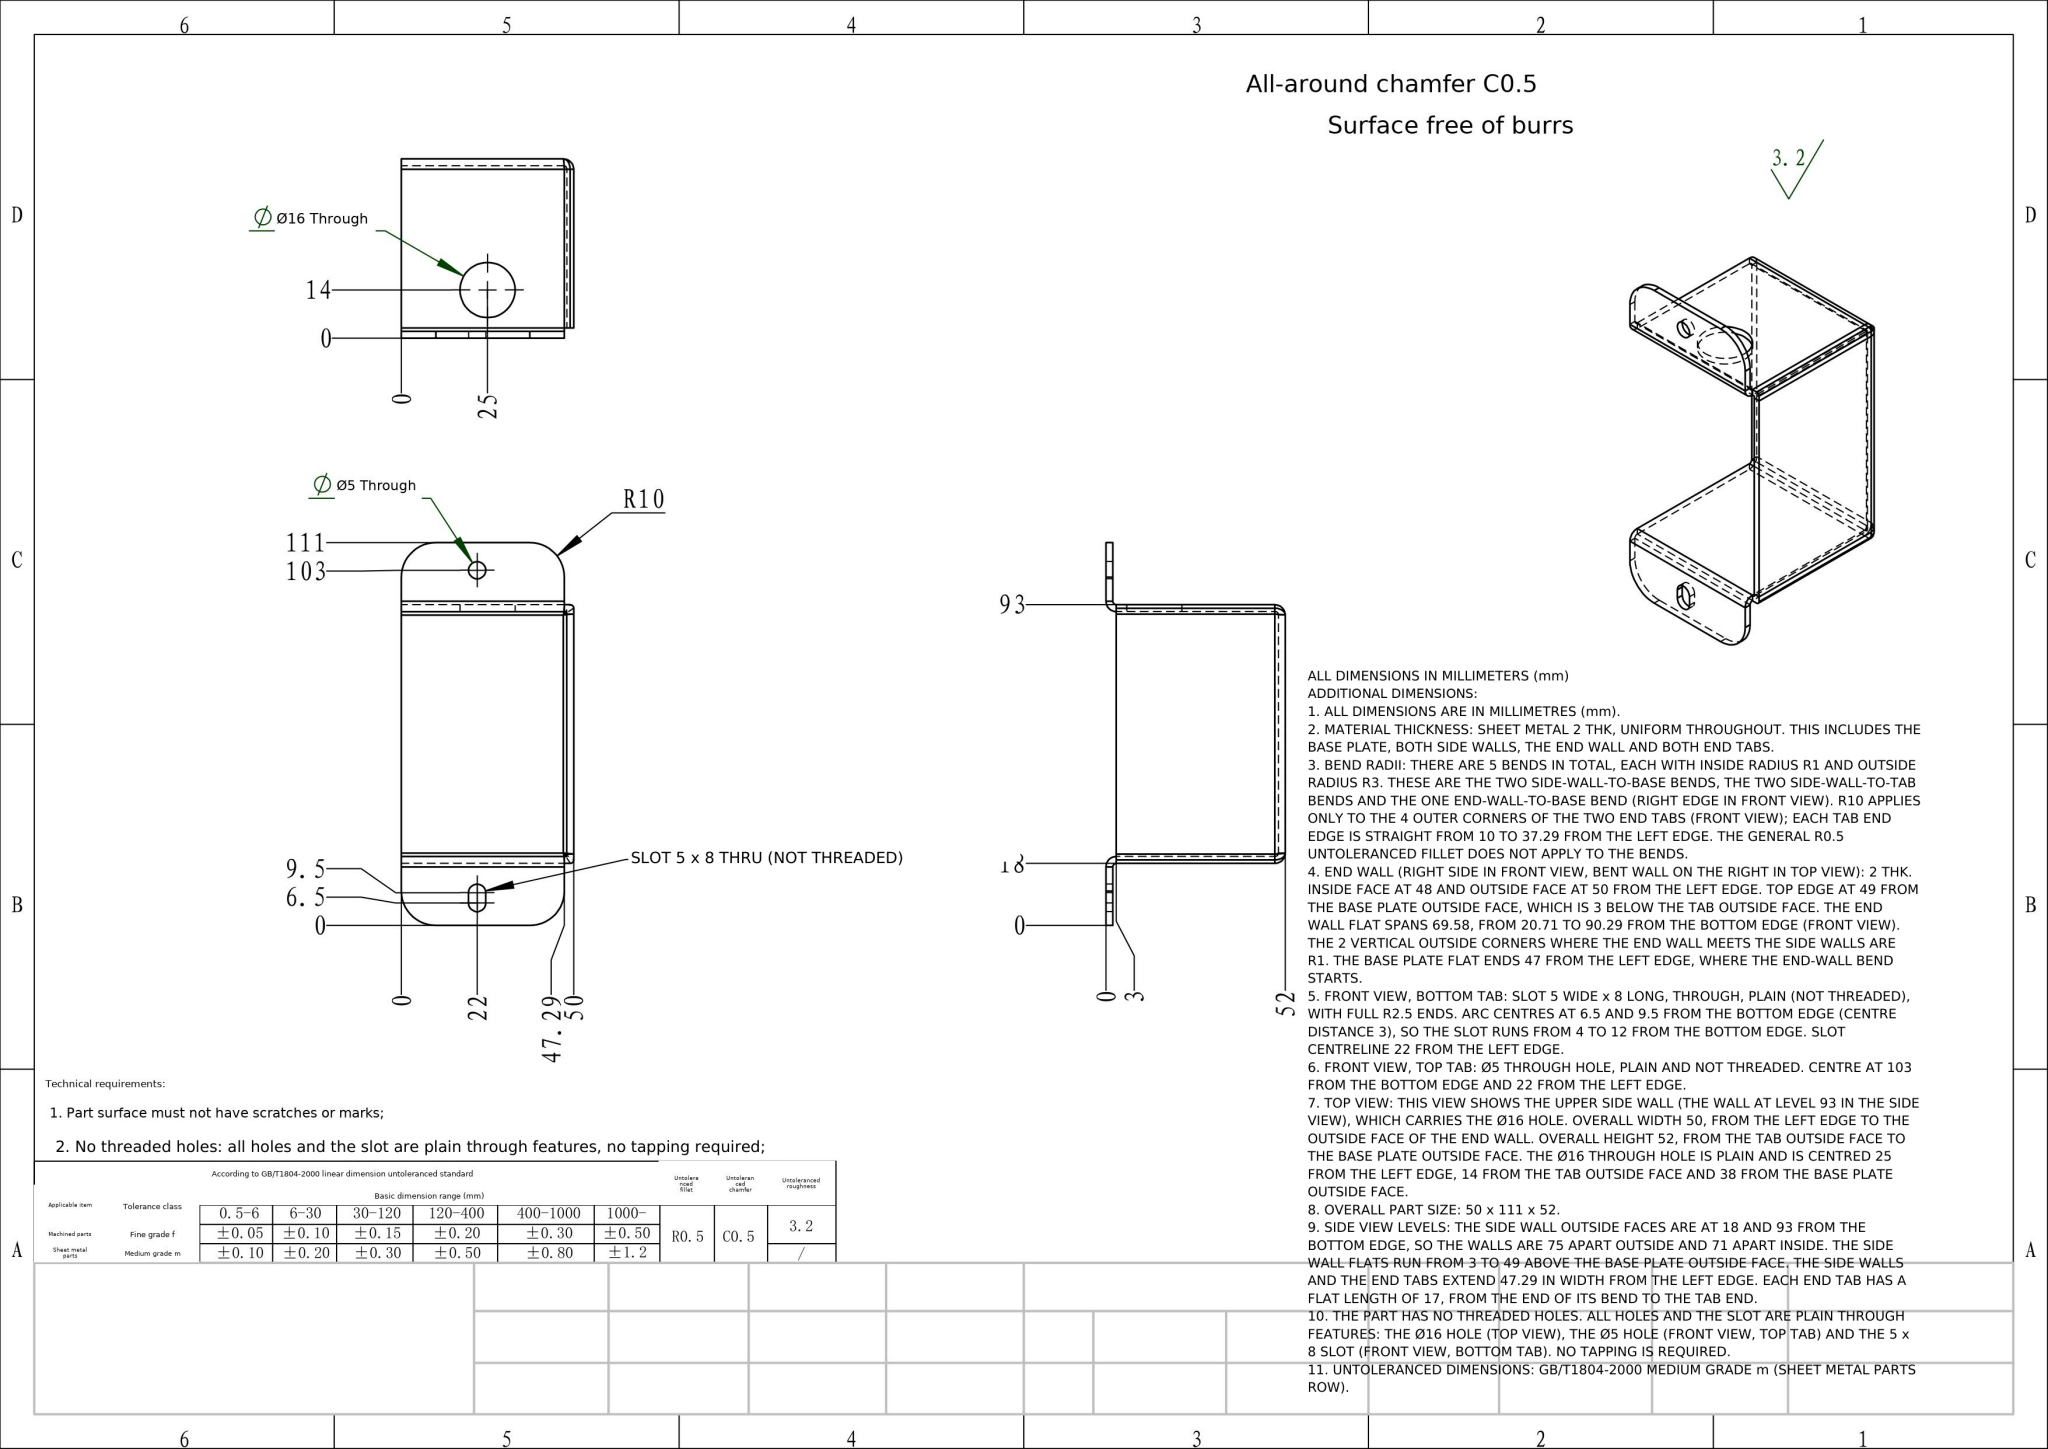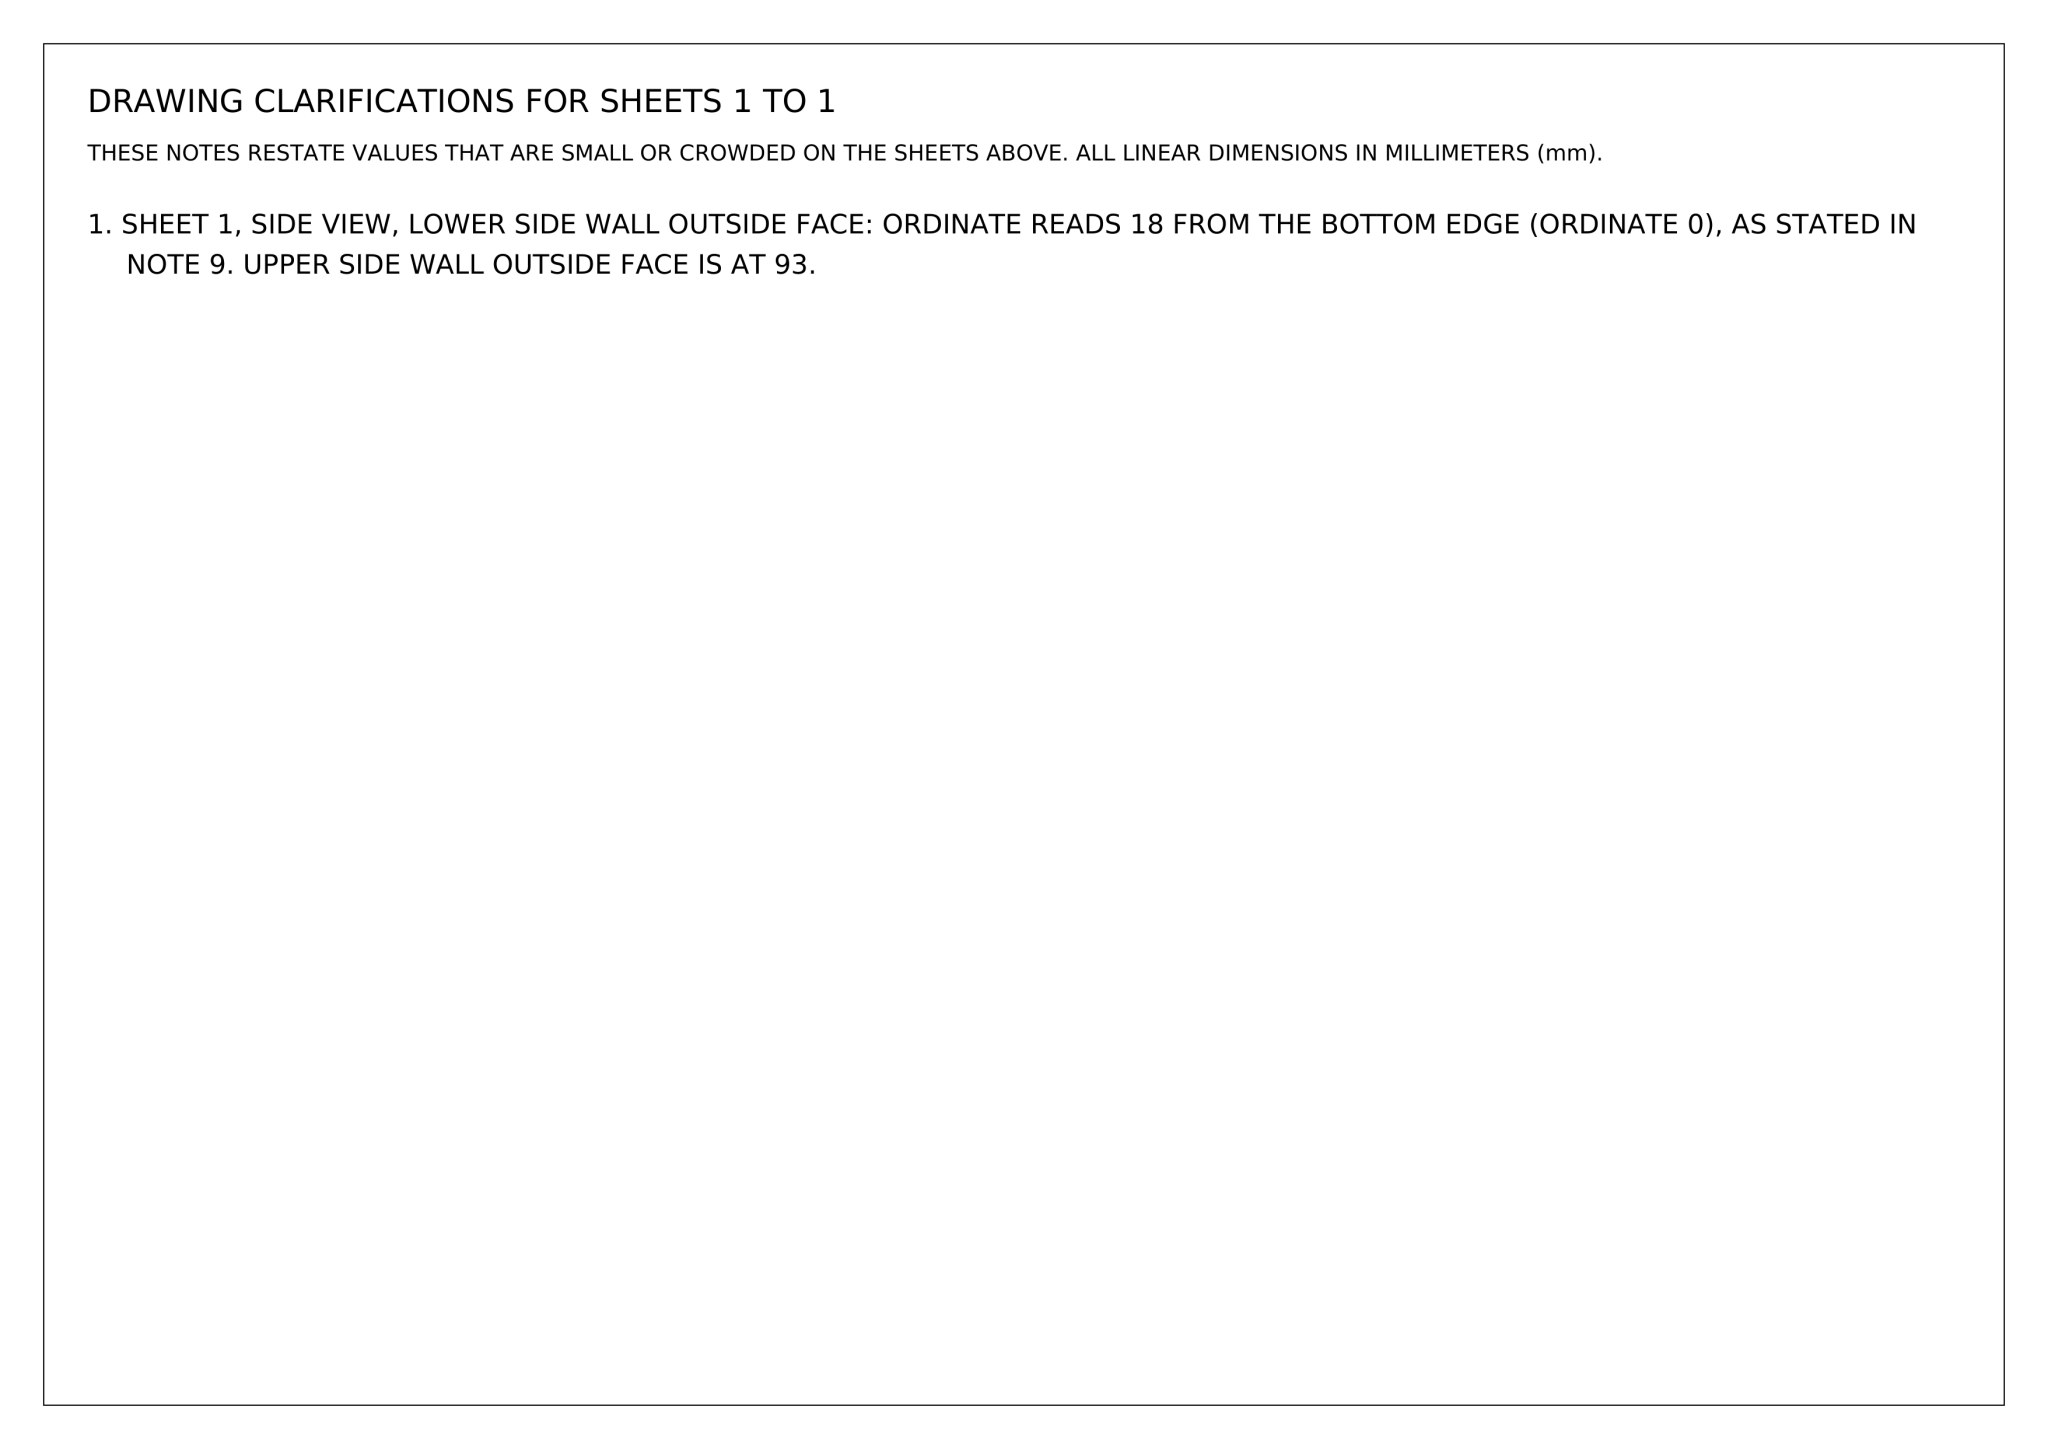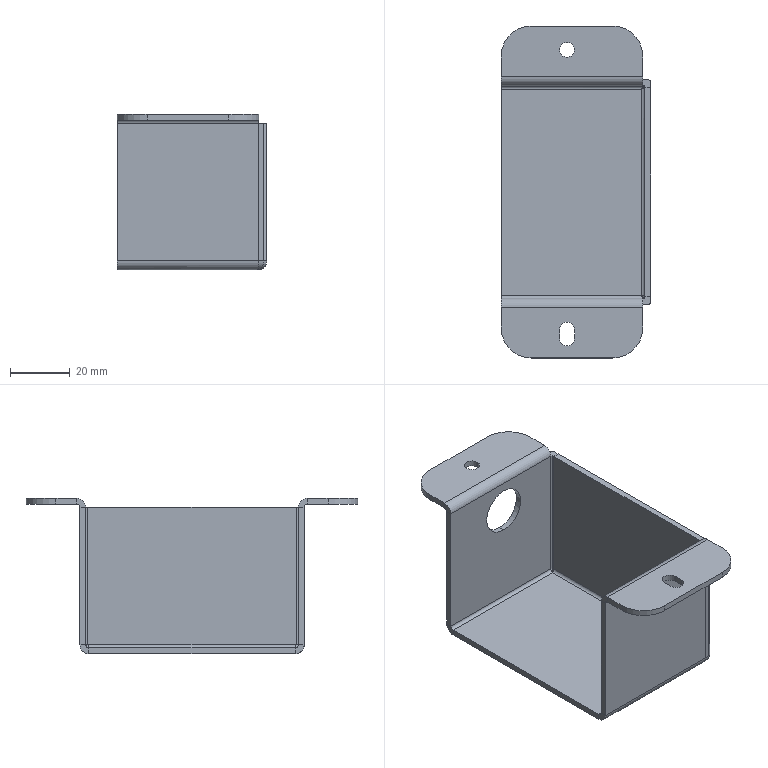Part | NX | mm | 1 solid | 72 faces | box 50 x 111 x 52 mm | volume 26384 mm3 | plane 40 | cylinder 22 | spline 10 | commonest cylinder face diameters 2 x7 6 x5 5 x4 20 x4 16 x2